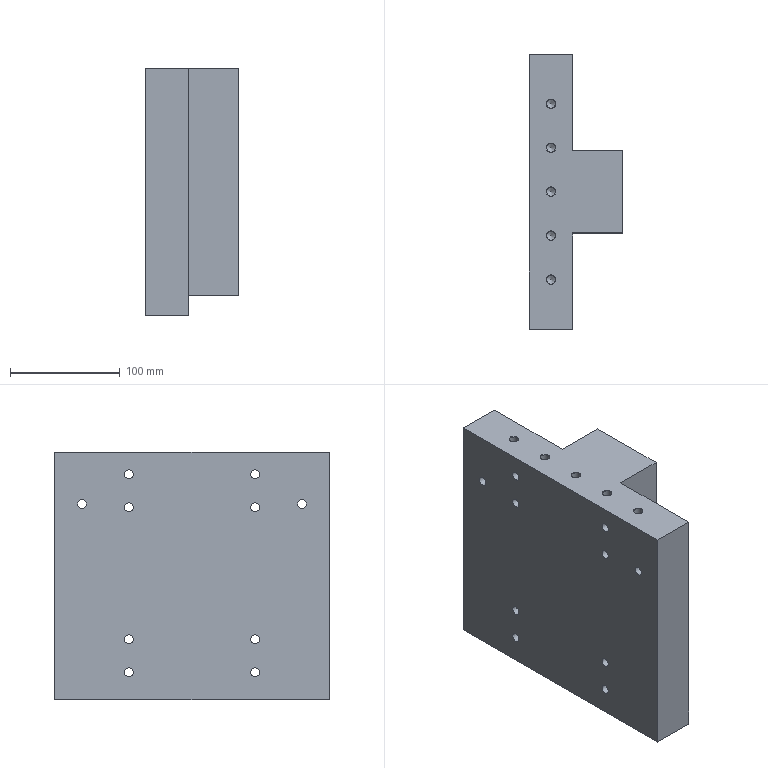Component | NX | SUPPORT_PLATE_2 | 1 solid | 50 faces | volume 2920778 mm3 | cylinder 20 | cone 20 | plane 10 | commonest cylinder face diameters 8 x20